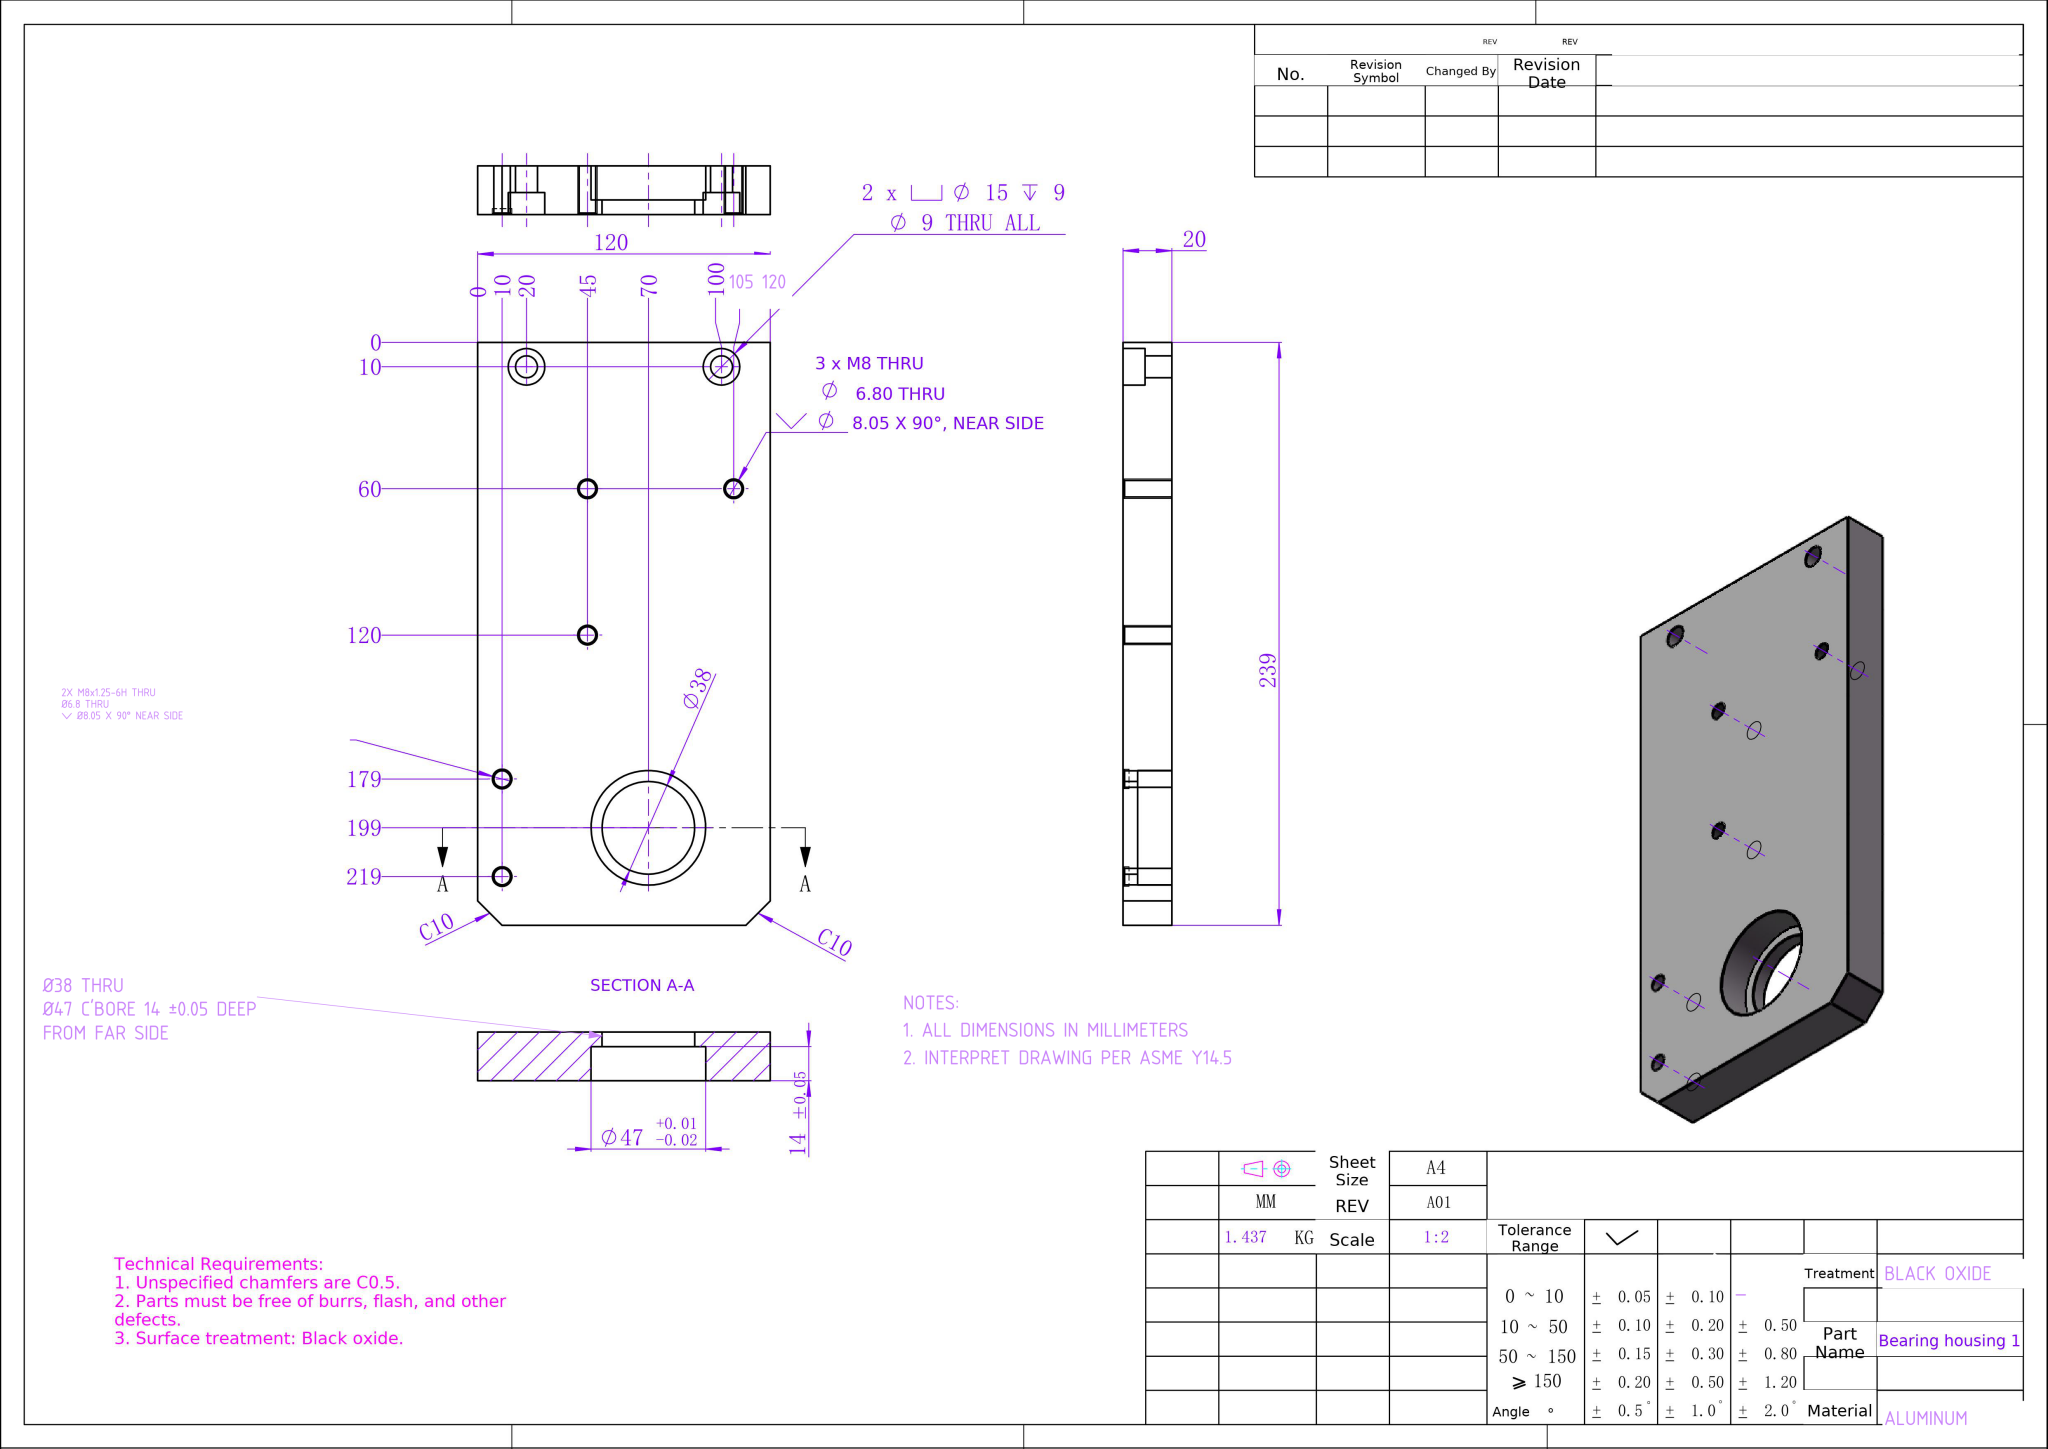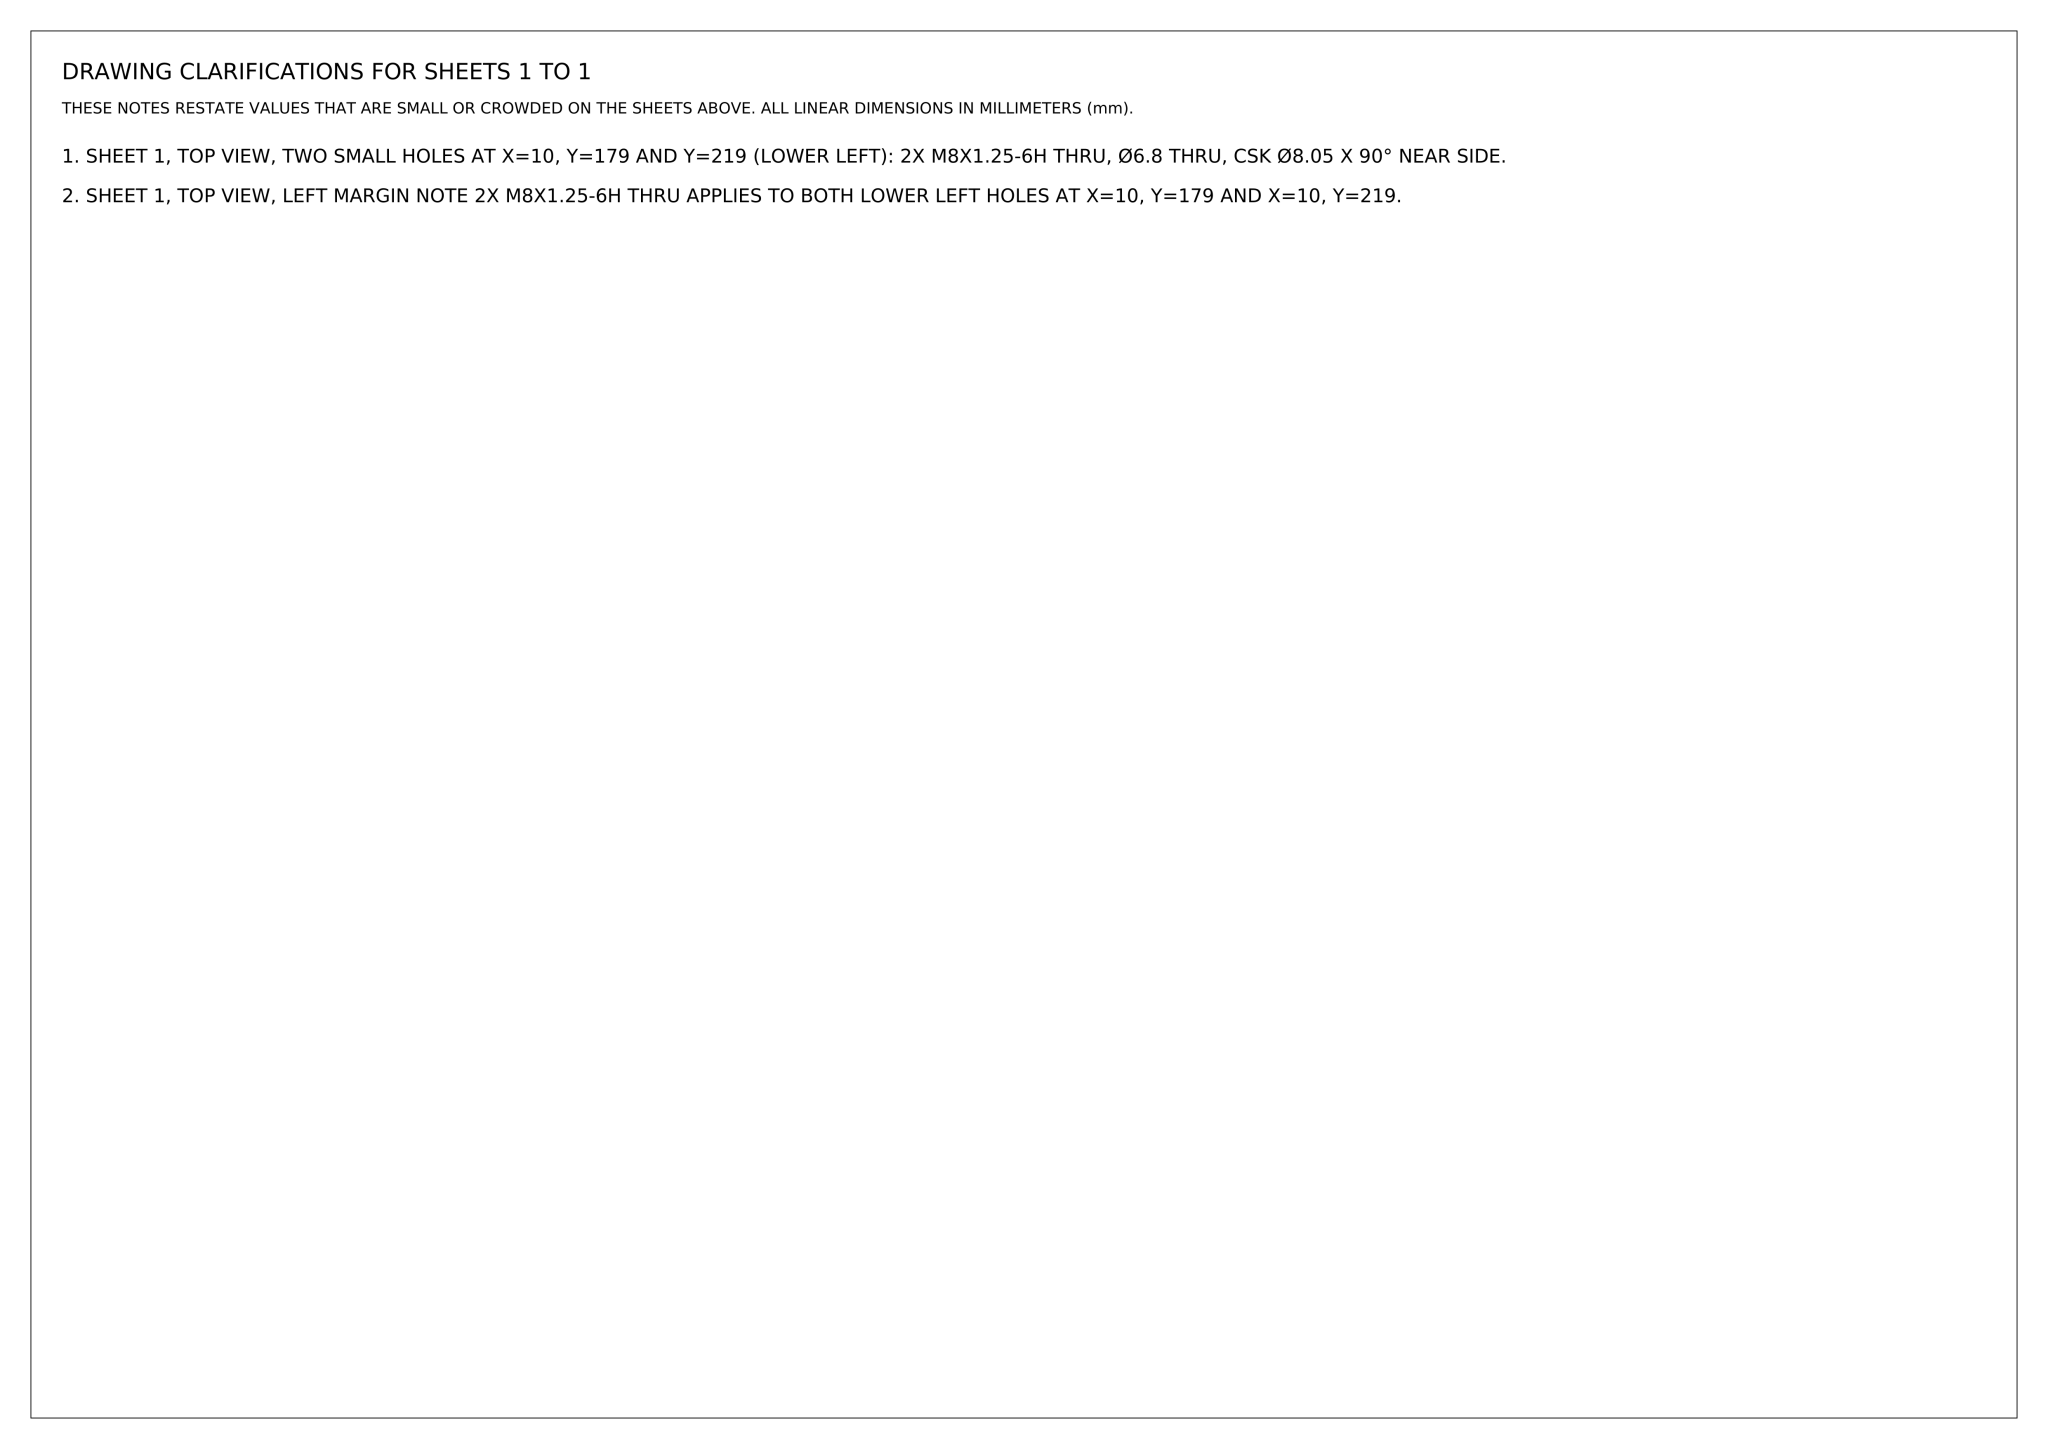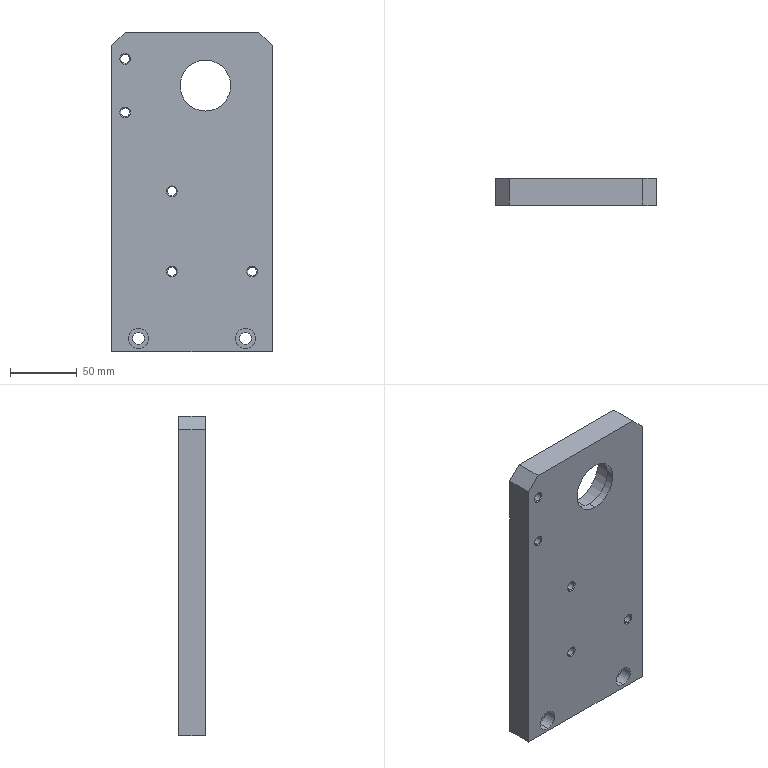Part | NX | mm | 1 solid | 43 faces | box 120 x 20 x 239 mm | volume 532272 mm3 | cylinder 22 | plane 11 | cone 10 | commonest cylinder face diameters 6.8 x10 9 x4 15 x4 38 x2 47 x2